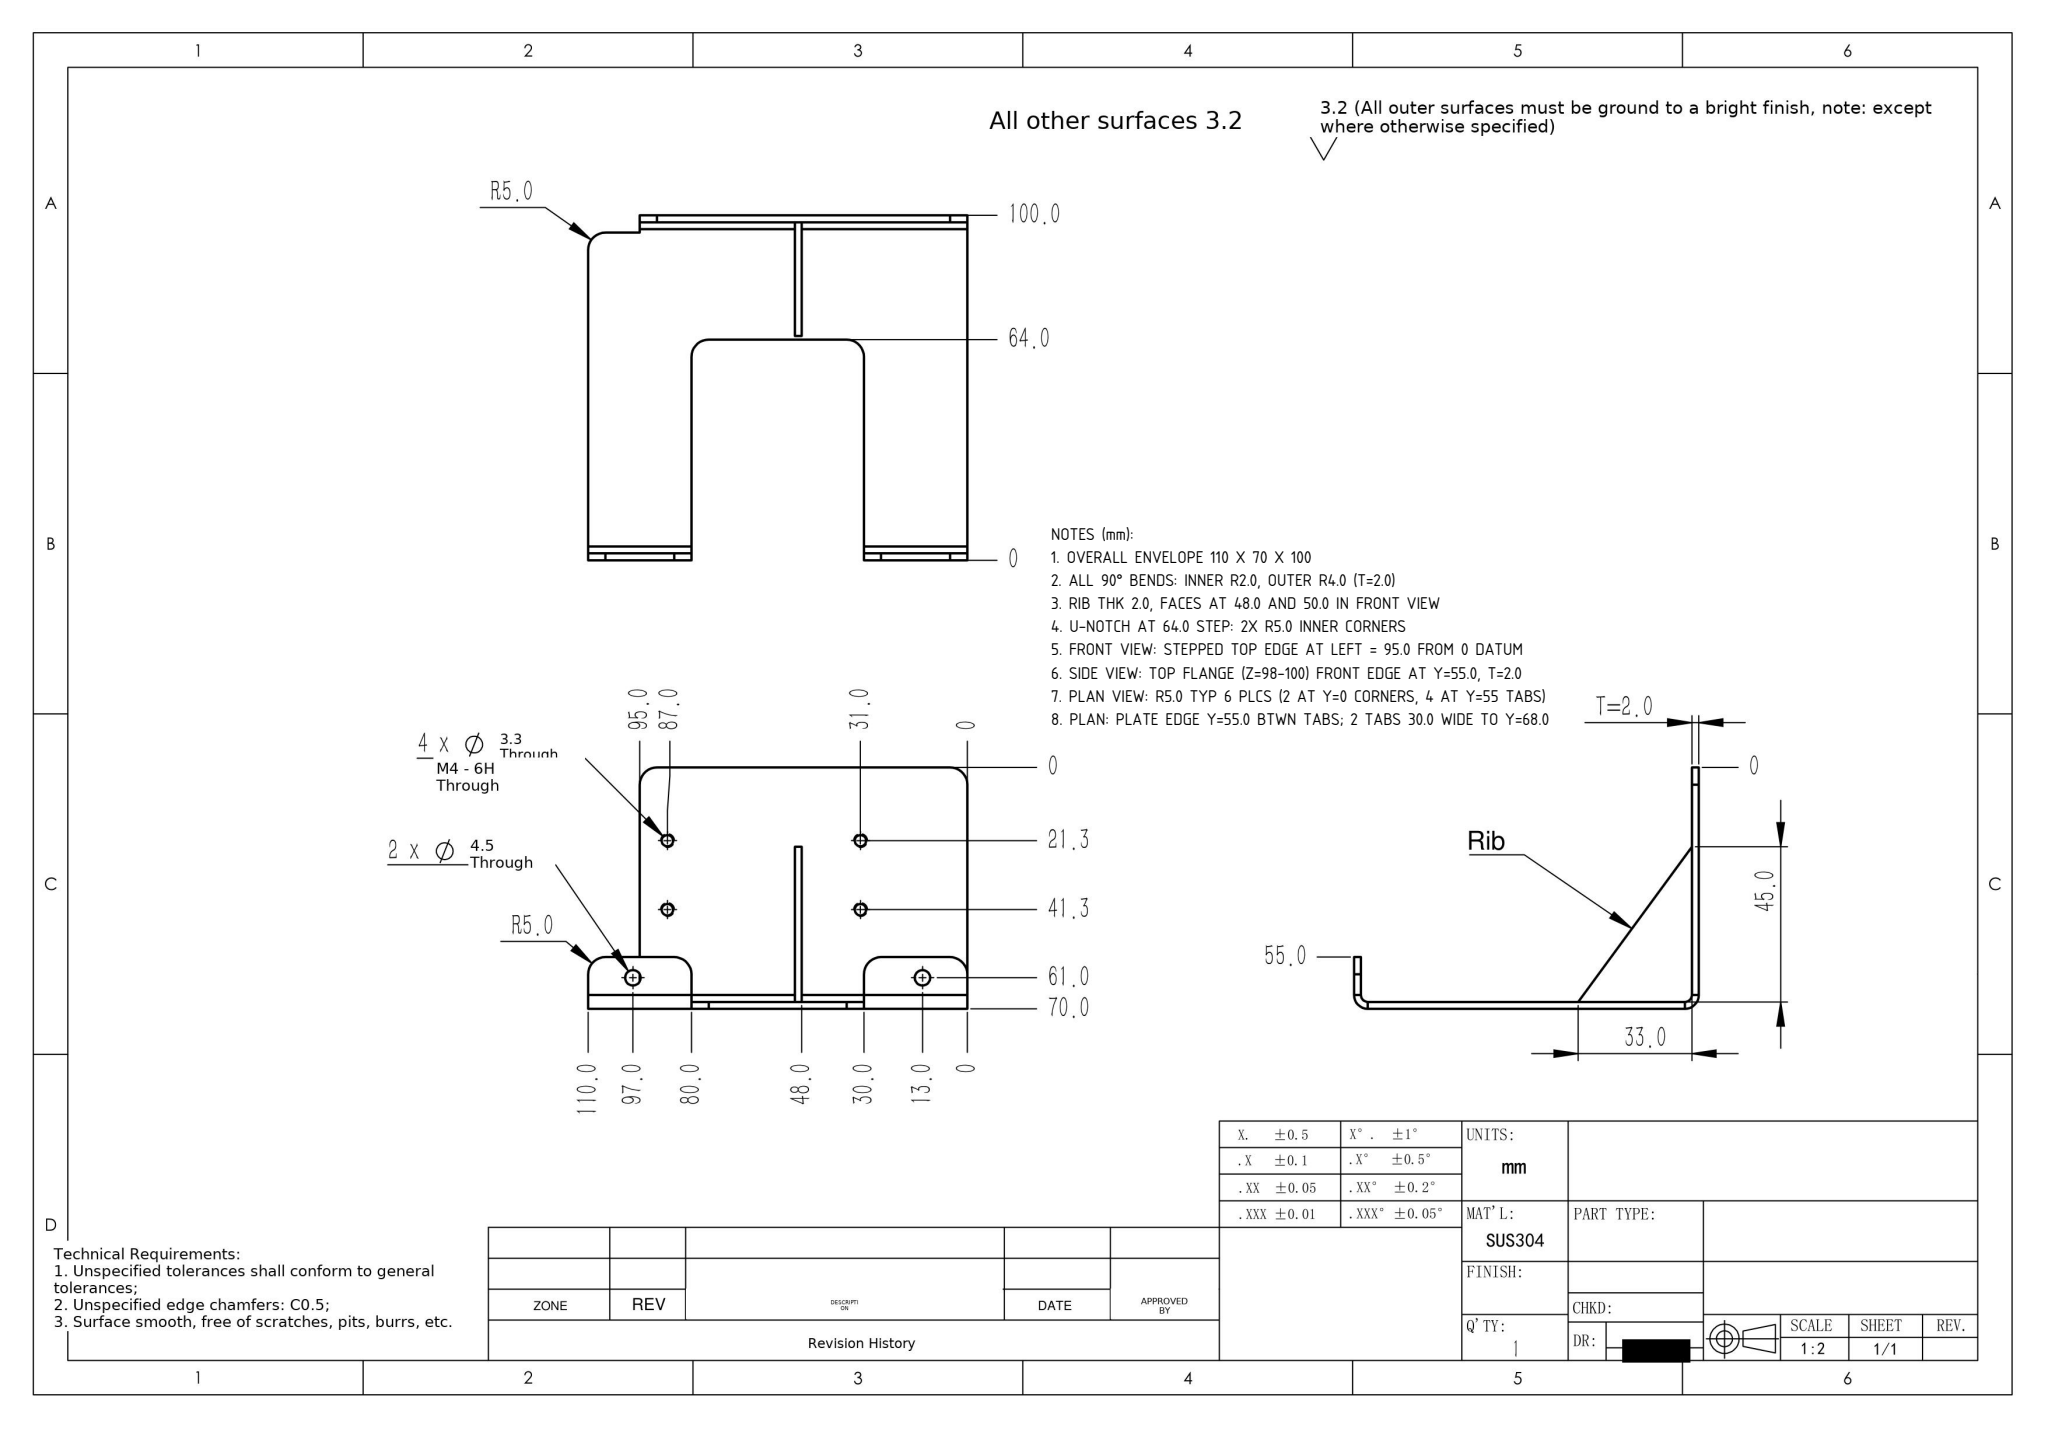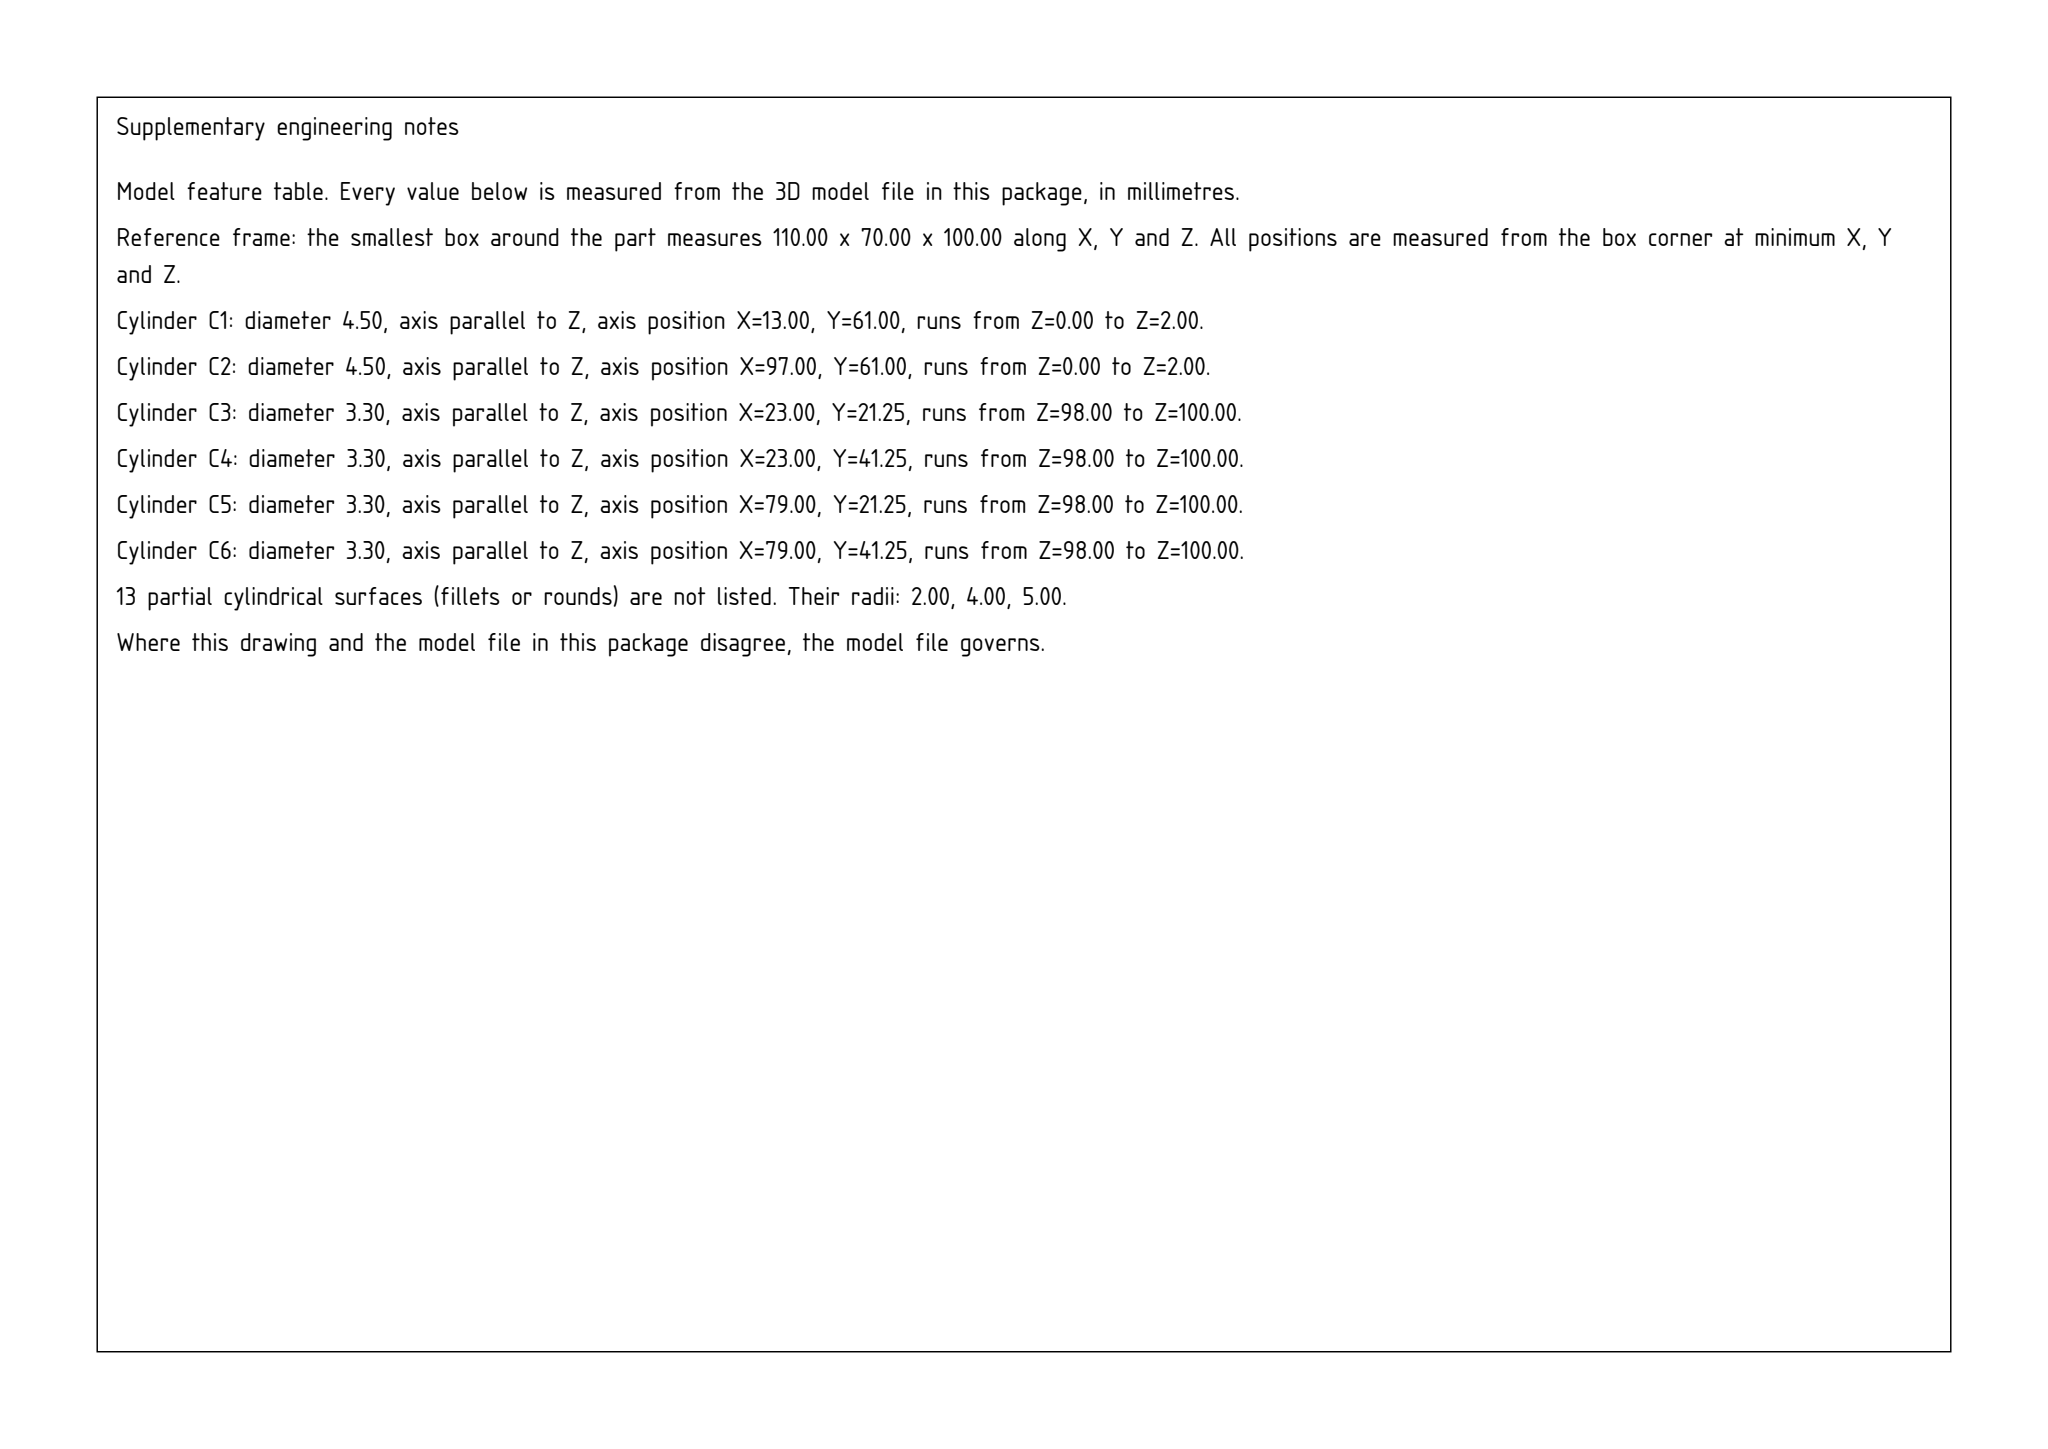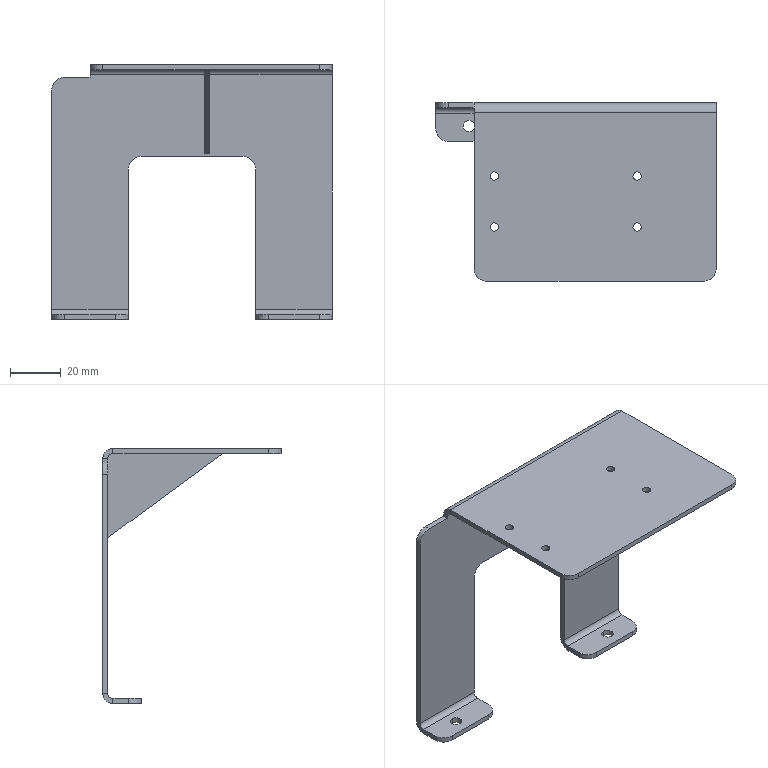Part | SolidWorks | mm | 1 solid | 61 faces | box 110 x 70 x 100 mm | volume 30828 mm3 | plane 33 | cylinder 28 | commonest cylinder face diameters 10 x9 3.3 x8 4.5 x4 4 x4 8 x3
Drawing notes:
OVERALL ENVELOPE 110 X 70 X 100 | from the solid: bbox_xyz [110.0, 70.0, 100.0]
ALL 90° BENDS: INNER R2.0, OUTER R4.0 (T=2.0) | from the solid: X-axis cyls Ø4.0 & Ø8.0 at (y66,z4) and (y66,z96): inner r2 / outer r4; T=2.0 from faces y68/y70, z0/z2, z98/z100
RIB THK 2.0, FACES AT 48.0 AND 50.0 IN FRONT VIEW | from the solid: X-normal planes at x=60.0 and x=62.0, 2.0 apart; 62.0 = 110-48.0 with right edge as 0 datum
U-NOTCH AT 64.0 STEP: 2X R5.0 INNER CORNERS | from the solid: Y-axis cyls Ø10.0 len 2.0 at (x35,z59) and (x75,z59) -> R5 fillets below z=64 notch
FRONT VIEW: STEPPED TOP EDGE AT LEFT = 95.0 FROM 0 DATUM | from the solid: z plane at 95.0 (1 face) vs top z=100.0; R5 (dia10 y-axis cyl at x=5,z=90) rounds corner x=0,z=95
SIDE VIEW: TOP FLANGE (Z=98-100) FRONT EDGE AT Y=55.0, T=2.0 | from the solid: z planes 98.0 and 100.0 with y plane 55.0 (2 faces); wall faces y=68.0/70.0 give 13.0 projection from inner face
PLAN VIEW: R5.0 TYP 6 PLCS (2 AT Y=0 CORNERS, 4 AT Y=55 TABS) | from the solid: dia10 z-axis cyls L=2: (20,5),(105,5) at y=0 edge; (5,60),(25,60),(85,60),(105,60) at y=55 tab junctions
PLAN: PLATE EDGE Y=55.0 BTWN TABS; 2 TABS 30.0 WIDE TO Y=68.0 | from the solid: x planes 0/30/80/110 define tabs; y plane 55.0 plate edge, y=68.0 wall inner face, y=70.0 wall back